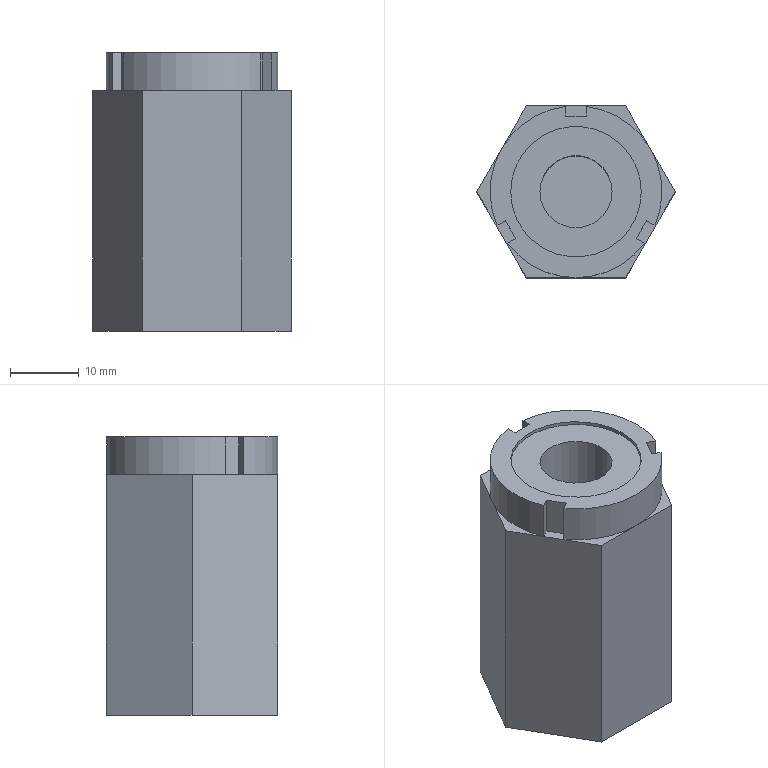CAM job | Mastercam | mm | 3 operations | part box 28.87 x 25 x 40.5
1. Contour (2D) | 14 - 2 平铣刀
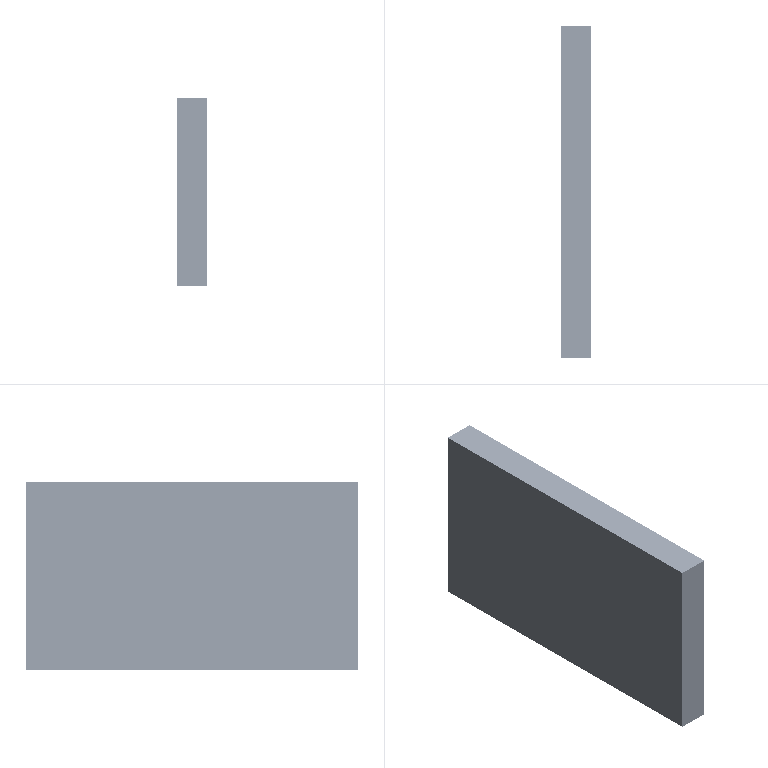2. Contour (2D) | 14 - 2 平铣刀
3. Peck Drill | 1 - 2.5 钻头